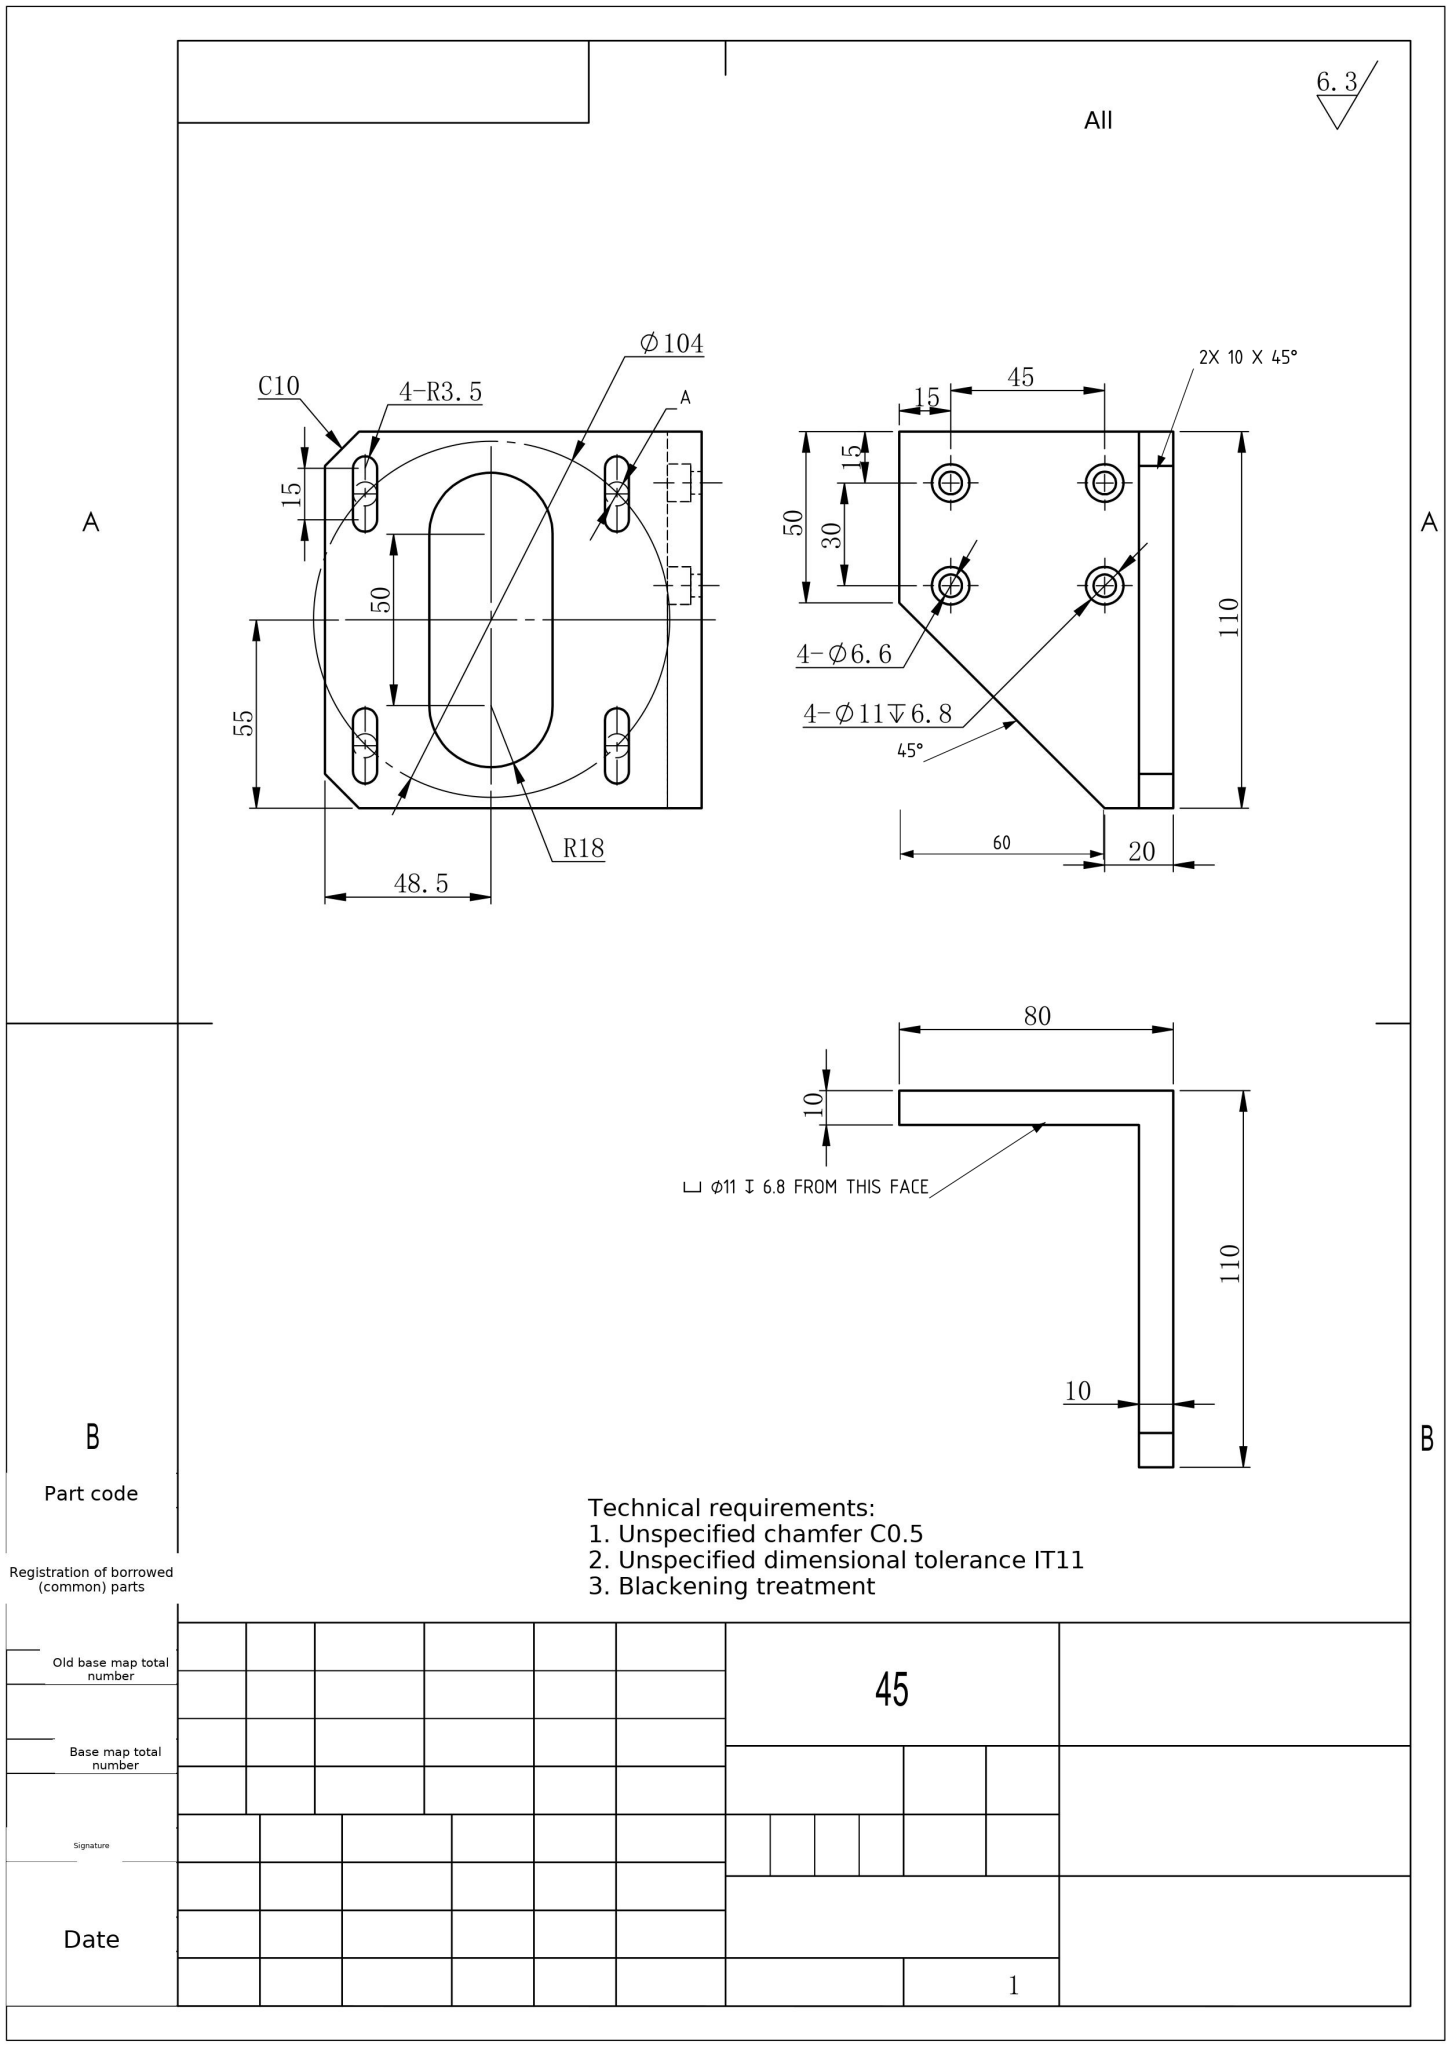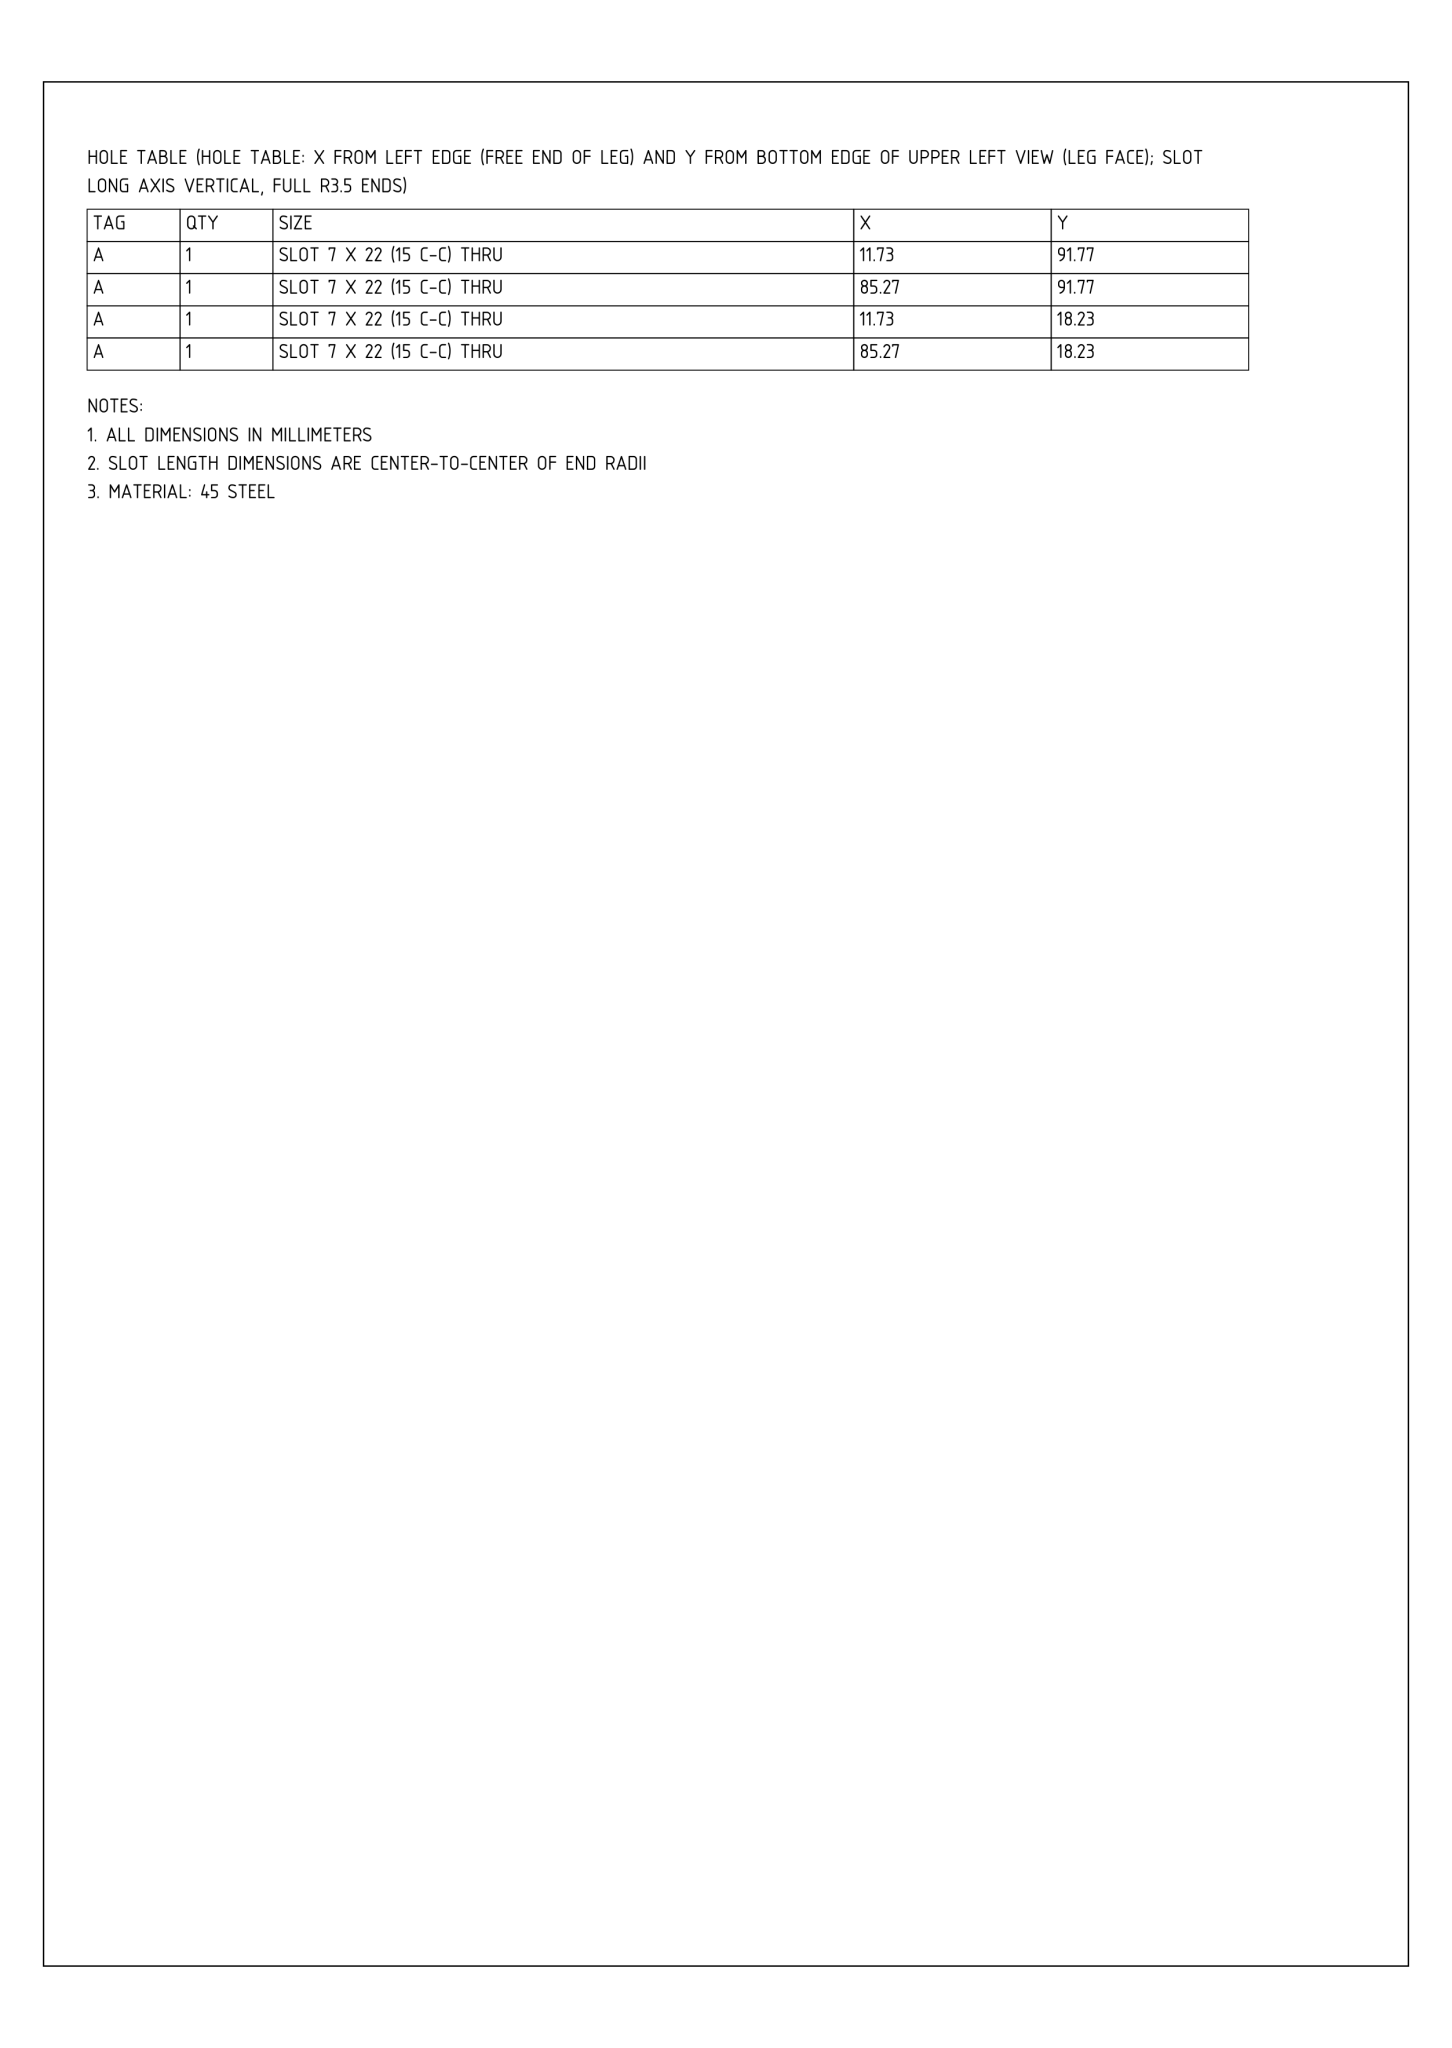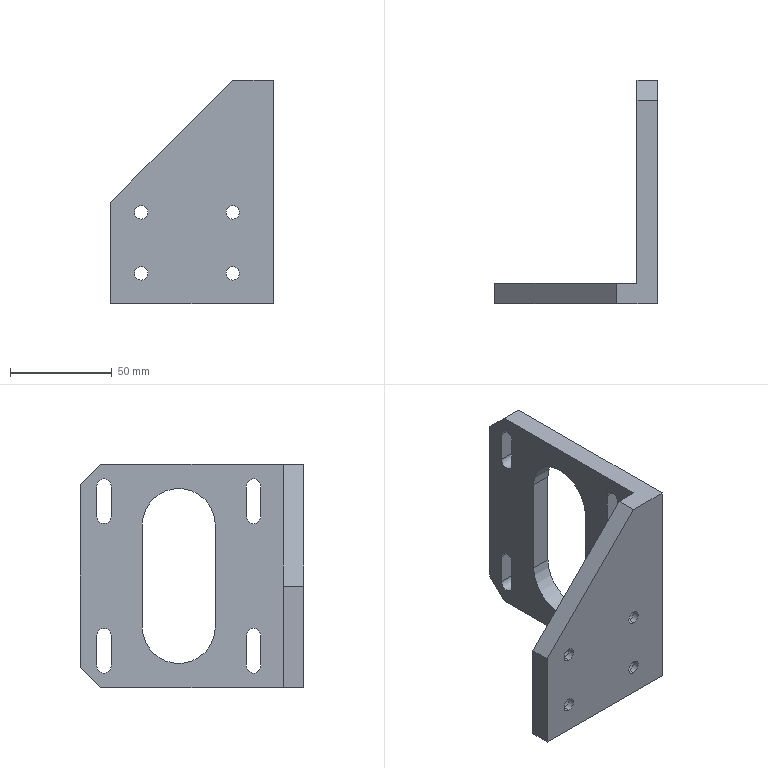Part | NX | mm | Right-Angle Slotted Oval-Aperture Bracket | 1 solid | 51 faces | box 80 x 110 x 110 mm | volume 142059 mm3 | cylinder 26 | plane 25 | commonest cylinder face diameters 11 x8 6.6 x8 7 x8 36 x2